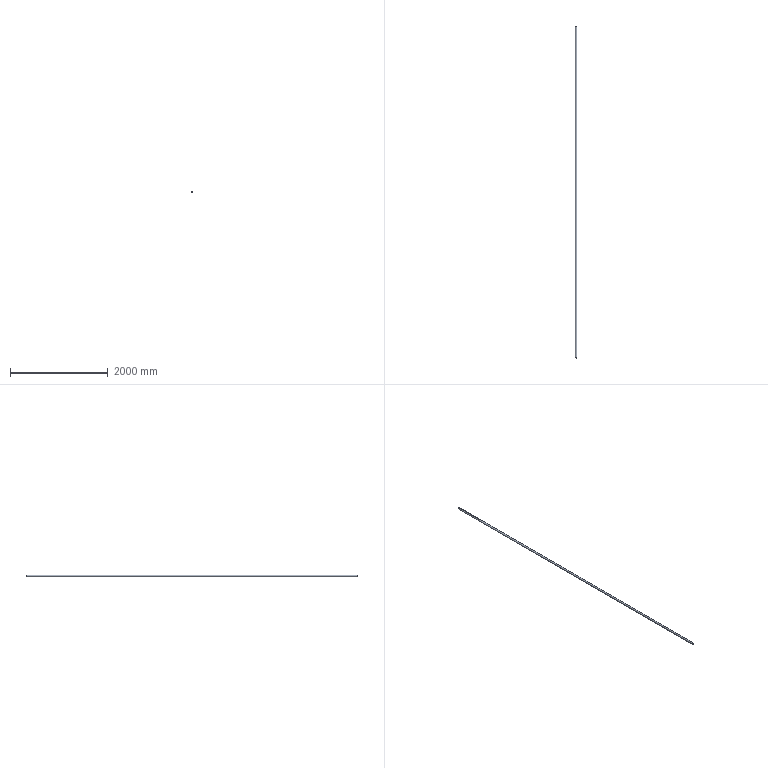Component | NX | 43_5 | 1 solid | 4 faces | volume 2278470 mm3 | cylinder 2 | plane 2 | commonest cylinder face diameters 34 x1 27 x1